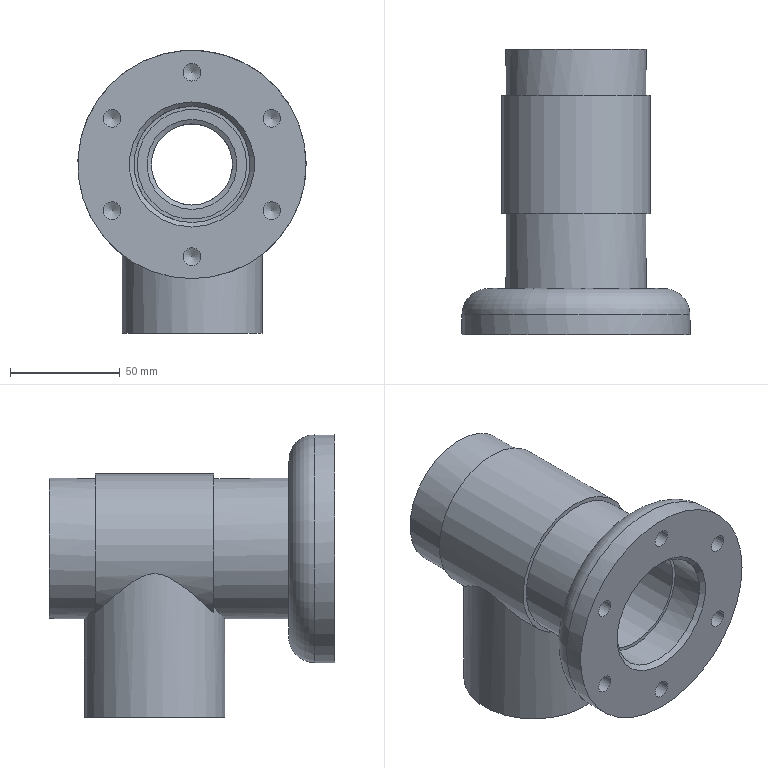Component | NX | VALVE_BODY | 1 solid | 41 faces | volume 388786 mm3 | cylinder 18 | plane 11 | cone 11 | torus 1 | commonest cylinder face diameters 8 x6 64 x3 40.5 x2 68 x1 104 x1 53 x1 50 x1 56 x1